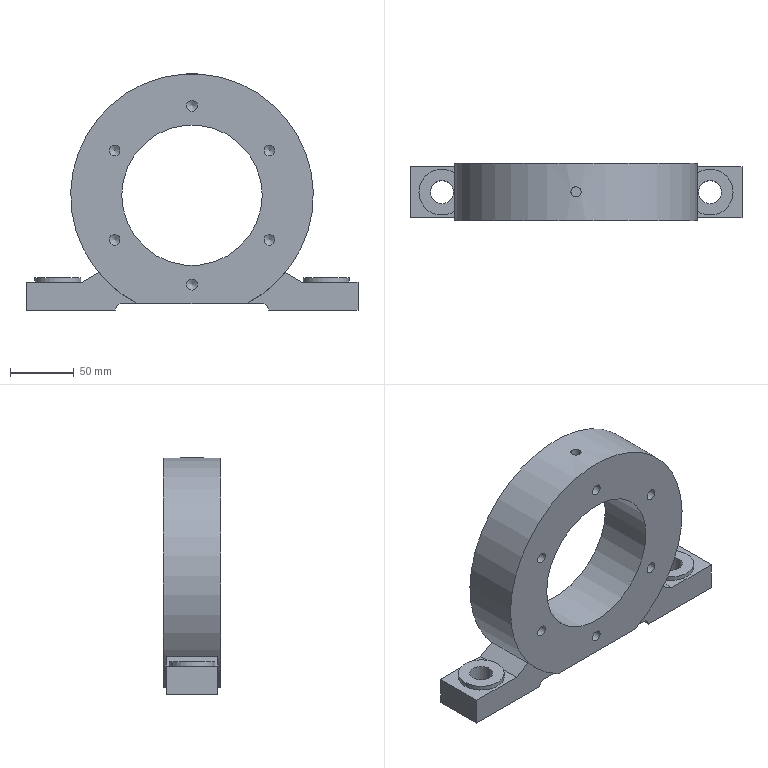Component | NX | BEARING_HOUSING | 1 solid | 50 faces | volume 939067 mm3 | cylinder 21 | plane 17 | cone 12 | commonest cylinder face diameters 8.5 x12 36 x2 18 x2 10 x2 190 x1 110 x1 8 x1